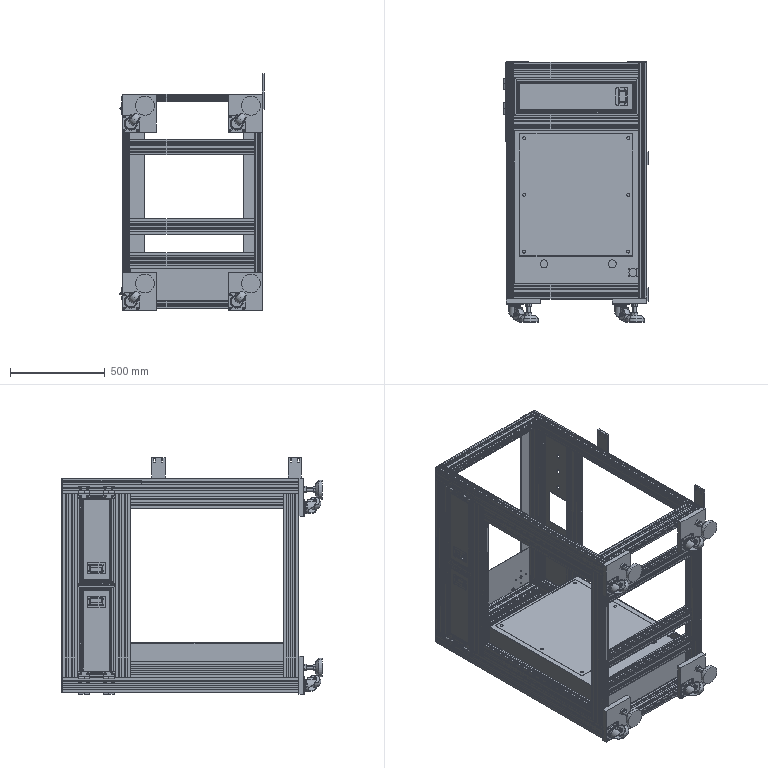Assembly | SolidWorks | mm | 62 component files | 97 solids | 3497 faces | box 762 x 1375 x 1252 mm | volume 33936133 mm3 | plane 2019 | cylinder 1170 | cone 148 | torus 128 | spline 24 | sphere 8 | commonest cylinder face diameters 8 x264 19 x216 6.8 x112 2 x60 10 x56 7 x56 5.5 x48 20 x32
Bill of materials:
10-15A | 1 |  | Long, narrow flat bar with small clipped corners and four through-holes arranged symmetrically along its length.
AluminumAlloyDoorAcrylicPlate(RearDoor) | 1 |  | Flat rectangular panel made of two stacked layers, with two hinge-like tabs along one short edge and a raised rounded-rectangle boss near the other end.
AluminumAlloyDoorAcrylicPlate(UpperSmallDoor) | 1 |  | Tall rectangular panel with hinge-like tabs at both short ends and two raised rounded-rectangle bosses near mid-height. It appears to be two panel sections stacked end to end.
EF4080-1080 | 1 |  | Straight extruded-style bar with a rectangular, multi-slot cross-section, shown standing vertically.
EF4080-500 | 4 |  | Long straight bar with the same kind of rectangular multi-slot cross-section, shown lying diagonally.
EF4080-550 | 2 |  | Long straight slotted bar whose cross-section looks the same as parts 3 and 4.
EF4080-920 | 5 |  | Straight slotted bar with a rectangular multi-cavity cross-section, shown standing vertically.
EF4080-940 | 8 |  | Long straight bar with a rectangular slotted cross-section, shown lying flat, with slots along the top face and the sides.
DistributionBox1 | 1 |  | Rectangular box-shaped body with plain faces. Holes are grouped near one edge of the top face, and there is one hole in a side face.
DistributionBoxDoor | 2 |  | Thin flat rectangular plate with no visible holes or features.
ElectricalControlPanel | 1 |  | Shallow square tray: a flat plate with a low upturned rim on all four edges and six small through-holes.
FrontSealingPlate | 1 |  | Long rectangular plate with short flanges bent along both long edges, forming a shallow channel.
TouchScreenPanel | 1 |  | Long, narrow rectangular flat plate. It has five small round through-holes on its centerline (three above and two below) and one rectangular through-cutout between the two groups.
CJH65bearing-322 | 4 |  | Solid cylinder whose length is roughly twice its diameter. Each end face shows a smaller concentric circular region, which suggests an edge chamfer/round, a shallow recess, or a boss.
CJH65body-322 | 4 |  | Compound fitting-like body. A cylindrical cup/socket with a large rounded closed end is joined at the side to an open, rectangular, channel-like clamp section. A bolt with hex head and nut is visible across the clamp section's slot.
CJH65swivel-322 | 4 |  | Square flat flange plate with rounded corners and four round through-holes, one near each corner. A central circular feature projects from one face, with tapered side walls and a flat top.
CJH65wheel-322 | 4 |  | Barrel-shaped body: a sphere-like or convex outer surface truncated by two parallel flat end faces, with a central cylindrical through-bore along the axis.
FBR20nut-322 | 4 |  | Hexagonal prism with a central round through-bore. The corners are chamfered on one end face, giving the curved chamfer arcs typical of a hex nut form.
pad1100-20-100pad1-322 | 4 |  | Disc-shaped base whose upper rim is conically tapered. On top sits a small hexagonal section, from which a long, slender cylindrical rod extends along the axis. The overall shape resembles a leveling foot.
WheelFixingPlate-322 | 4 |  | Thick, nearly square rectangular plate with five round through-holes: one larger hole near an upper corner region and four smaller holes in a rectangular/square pattern toward the opposite side.
30-42A | 1 |  | Very thin, large rectangular sheet with many round through-holes of several sizes. These include small holes near the edges and corners, two medium holes, and a cluster of one central hole surrounded by four tiny holes.
30-43A | 1 |  | Long, very thin rectangular strip with four small round through-holes, evenly spaced in a line near one long edge.
30-44A | 1 |  | Long, very thin rectangular strip with four small round through-holes, evenly spaced in a line near one long edge (the side opposite to the similar strip in the set).
30-71A | 2 |  | Thick rectangular plate. Two parallel elongated slots with rounded ends run lengthwise at one end, and four round through-holes form a two-by-two pattern at the other end.
Mates:
1. coincident | 30-01A-1/EF4080-920-4 face at (-423.23, 712.155, -40) dir (0, 1, 0) | 30-43A-1 face at (-447.43, 712.155, 40) dir (0, -1, 0)
2. coincident | 30-01A-1/EF4080-500-1 face at (-447.43, 712.155, 40) dir (0, 0, 1) | 30-43A-1 face at (-327.43, 712.155, 40) dir (0, 0, 1)
3. coincident | 30-01A-1/EF4080-500-1 face at (-447.43, 712.155, 40) dir (-1, 0, 0) | 30-43A-1 face at (-447.43, 712.155, 40) dir (-1, 0, 0)
4. coincident | 30-01A-1/EF4080-920-3 face at (276.77, 712.155, -40) dir (0, 1, 0) | 30-44A-1 face at (192.57, 712.155, 40) dir (0, -1, 0)
5. coincident | 30-01A-1/EF4080-500-2 face at (292.57, 712.155, -15.8) dir (1, 0, 0) | 30-44A-1 face at (292.57, 712.155, 40) dir (1, 0, 0)
6. coincident | 30-01A-1/EF4080-500-2 face at (276.77, 712.155, 40) dir (0, 0, 1) | 30-44A-1 face at (292.57, 712.155, 40) dir (0, 0, 1)
7. coincident | 30-01A-1/EF4080-940-6 face at (-407.43, 712.155, -1074.2) dir (0, 1, 0) | 30-42A-1 face at (-447.43, 712.155, -828) dir (0, -1, 0)
8. coincident | 30-01A-1/EF4080-500-4 face at (292.57, 712.155, -1090) dir (1, 0, 0) | 30-42A-1 face at (292.57, 714.155, -1090) dir (1, 0, 0)
9. coincident | 30-01A-1/EF4080-500-4 face at (276.77, 712.155, -1090) dir (0, 0, -1) | 30-42A-1 face at (-447.43, 714.155, -1090) dir (0, 0, -1)
10. coincident | 30-01A-1/EF4080-500-2 face at (292.57, 712.155, -15.8) dir (1, 0, 0) | 30-71A-1 face at (292.57, -480.845, -40) dir (-1, 0, 0)
11. coincident | 30-01A-1/EF4080-500-2 face at (276.77, 712.155, -40) dir (0, 0, -1) | 30-71A-1 face at (292.57, -480.845, -40) dir (0, 0, -1)
12. distance | 30-01A-1/EF4080-920-2 face at (276.77, -537.845, -40) dir (0, -1, 0) | 30-71A-1 face at (292.57, -550.845, 150) dir (0, -1, 0)
13. coincident | 30-01A-1/EF4080-500-1 face at (-447.43, 712.155, 15.8) dir (-1, 0, 0) | 10-15A-1 face at (-447.43, 712.155, 30) dir (1, 0, 0)
14. coincident | 30-01A-1/EF4080-940-7 face at (-407.43, 712.155, 40) dir (0, 1, 0) | 10-15A-1 face at (-449.43, 712.155, 30) dir (0, 1, 0)
15. distance | 30-01A-1/EF4080-500-1 face at (-447.43, 712.155, 40) dir (0, 0, 1) | 10-15A-1 face at (-449.43, 292.155, 10) dir (0, 0, -1)
16. coincident | EF4080-500-1 face at (-122.809, 641.189, -15.8) dir (1, 0, 0) | EF4080-940-1 face at (-122.809, -533.311, 20) dir (-1, 0, 0)
17. coincident | EF4080-500-1 face at (-138.609, 641.189, -40) dir (0, 0, -1) | EF4080-920-1 face at (-142.809, -604.311, -40) dir (0, 0, 1)
18. coincident | EF4080-500-1 face at (-122.809, 641.189, -40) dir (1, 0, 0) | EF4080-920-1 face at (-122.809, -553.011, -40) dir (1, 0, 0)
19. coincident | EF4080-500-1 face at (-142.809, -608.811, 35.5) dir (0, -1, 0) | EF4080-920-1 face at (-138.609, -608.811, -40) dir (0, -1, 0)
20. coincident | EF4080-500-1 face at (-138.609, 641.189, 40) dir (0, 0, 1) | EF4080-940-1 face at (-122.809, -553.011, 40) dir (0, 0, 1)
21. coincident | EF4080-500-1 face at (-142.809, -608.811, 35.5) dir (0, -1, 0) | EF4080-940-1 face at (-122.809, -608.811, 40) dir (0, -1, 0)
22. coincident | EF4080-500-3 face at (-122.809, 641.189, -1065.8) dir (1, 0, 0) | EF4080-940-5 face at (-122.809, -533.311, -1070) dir (-1, 0, 0)
23. coincident | EF4080-500-3 face at (-142.809, -608.811, -1014.5) dir (0, -1, 0) | EF4080-940-5 face at (-122.809, -608.811, -1050) dir (0, -1, 0)
24. coincident | EF4080-500-3 face at (-138.609, 641.189, -1090) dir (0, 0, -1) | EF4080-940-5 face at (-122.809, -584.611, -1090) dir (0, 0, -1)
25. coincident | EF4080-500-2 face at (561.391, 641.189, -40) dir (0, 0, -1) | EF4080-920-2 face at (557.191, -604.311, -40) dir (0, 0, 1)
26. coincident | EF4080-500-2 face at (577.191, 641.189, -40) dir (1, 0, 0) | EF4080-920-2 face at (577.191, -608.811, -40) dir (1, 0, 0)
27. coincident | EF4080-500-2 face at (557.191, -608.811, 35.5) dir (0, -1, 0) | EF4080-920-2 face at (561.391, -608.811, -40) dir (0, -1, 0)
28. coincident | EF4080-920-2 face at (537.191, -608.811, -40) dir (0, -1, 0) | Wheel-322-1/WheelFixingPlate-322-1 face at (577.191, -608.811, 40) dir (0, 1, 0)
29. coincident | EF4080-920-2 face at (577.191, -553.011, -40) dir (1, 0, 0) | Wheel-322-1/WheelFixingPlate-322-1 face at (577.191, -608.811, 40) dir (1, 0, 0)
30. coincident | EF4080-940-1 face at (-122.809, -553.011, 40) dir (0, 0, 1) | Wheel-322-1/WheelFixingPlate-322-1 face at (397.191, -608.811, 40) dir (0, 0, 1)
31. coincident | EF4080-920-2 face at (537.191, -584.611, -40) dir (-1, 0, 0) | EF4080-940-9 face at (537.191, -548.811, -273.5) dir (1, 0, 0)
32. coincident | EF4080-920-2 face at (537.191, -528.811, -40) dir (0, 1, 0) | EF4080-940-9 face at (-122.809, -528.811, -253.8) dir (0, 1, 0)
33. distance | EF4080-500-2 face at (537.191, 641.189, -40) dir (0, 0, -1) | EF4080-940-9 face at (-122.809, -528.811, -198) dir (0, 0, 1)
34. coincident | EF4080-500-2 face at (577.191, 641.189, -15.8) dir (1, 0, 0) | TouchScreenPanel-1 face at (577.191, 361.189, -40) dir (1, 0, 0)
35. coincident | EF4080-500-2 face at (561.391, 641.189, -40) dir (0, 0, -1) | TouchScreenPanel-1 face at (575.191, 361.189, -40) dir (0, 0, 1)
36. coincident | EF4080-920-3 face at (561.391, 561.189, -40) dir (0, -1, 0) | TouchScreenPanel-1 face at (575.191, 561.189, -40) dir (0, 1, 0)
37. coincident | EF4080-920-4 face at (-162.809, 561.189, -40) dir (-1, 0, 0) | AluminumAlloyDoorAcrylicPlate(UpperSmallDoor)-1 face at (-162.809, 531.189, -524) dir (-1, 0, 0)
38. coincident | EF4080-920-4 face at (-162.809, 561.189, -40) dir (0, -1, 0) | AluminumAlloyDoorAcrylicPlate(UpperSmallDoor)-1 face at (-162.809, 561.189, -524) dir (0, 1, 0)
39. coincident | EF4080-500-1 face at (-138.609, 641.189, -40) dir (0, 0, -1) | AluminumAlloyDoorAcrylicPlate(UpperSmallDoor)-1 face at (-154.059, 561.189, -40) dir (0, 0, 1)
40. coincident | EF4080-940-6 face at (-122.809, 561.189, -1090) dir (0, 0, -1) | AluminumAlloyDoorAcrylicPlate(RearDoor)-1 face at (537.191, 361.189, -1090) dir (0, 0, -1)
41. coincident | EF4080-940-10 face at (-122.809, -528.811, -673.8) dir (0, 1, 0) | FrontSealingPlate-1 face at (537.191, -528.811, -1050) dir (0, 1, 0)
42. coincident | EF4080-920-1 face at (-122.809, -553.011, -40) dir (1, 0, 0) | FrontSealingPlate-1 face at (-122.809, -530.811, -1050) dir (-1, 0, 0)
43. coincident | FrontSealingPlate-1 face at (537.191, -548.811, -878) dir (0, 0, 1) | EF4080-940-12 face at (-122.809, -553.011, -878) dir (0, 0, -1)
44. coincident | EF4080-500-3 face at (-162.809, 641.189, -1010) dir (0, 0, 1) | EF4080-550-1 face at (-162.809, 281.189, -1010) dir (0, 0, -1)
45. coincident | EF4080-500-1 face at (-138.609, 641.189, -40) dir (0, 0, -1) | EF4080-1080-1 face at (-142.809, 356.689, -40) dir (0, 0, 1)
46. coincident | EF4080-500-1 face at (-162.809, 641.189, 15.8) dir (-1, 0, 0) | EF4080-1080-1 face at (-162.809, 336.989, -1010) dir (-1, 0, 0)
47. coincident | EF4080-1080-1 face at (-162.809, 361.189, -1010) dir (0, 1, 0) | AluminumAlloyDoorAcrylicPlate(UpperSmallDoor)-1 face at (-161.559, 361.189, -524) dir (0, -1, 0)
48. coincident | EF4080-500-1 face at (-162.809, 641.189, -40) dir (0, 0, -1) | EF4080-550-2 face at (-162.809, 281.189, -40) dir (0, 0, 1)
49. coincident | EF4080-1080-1 face at (-162.809, 296.989, -1010) dir (-1, 0, 0) | EF4080-550-2 face at (-162.809, 281.189, -64.2) dir (-1, 0, 0)
50. coincident | EF4080-1080-1 face at (-138.609, 281.189, -1010) dir (0, -1, 0) | EF4080-550-2 face at (-142.809, 281.189, -44.5) dir (0, 1, 0)
51. coincident | EF4080-500-3 face at (-162.809, 641.189, -1034.2) dir (-1, 0, 0) | EF4080-550-1 face at (-162.809, 281.189, -954.2) dir (-1, 0, 0)
52. coincident | EF4080-920-1 face at (-162.809, -528.811, -40) dir (0, 1, 0) | EF4080-550-1 face at (-142.809, -528.811, -934.5) dir (0, -1, 0)
53. coincident | EF4080-940-12 face at (-122.809, -528.811, -853.8) dir (0, 1, 0) | ElectricalControlBox-1/DistributionBox1-1 face at (537.191, -528.811, -1090) dir (0, -1, 0)
54. coincident | EF4080-500-4 face at (537.191, 641.189, -1034.2) dir (-1, 0, 0) | ElectricalControlBox-1/DistributionBox1-1 face at (537.191, 281.189, -1090) dir (1, 0, 0)
55. coincident | EF4080-500-4 face at (537.191, 641.189, -1090) dir (0, 0, -1) | ElectricalControlBox-1/DistributionBoxDoor-1 face at (526.191, -517.811, -1090) dir (0, 0, -1)
56. coincident | EF4080-500-4 face at (537.191, 641.189, -1034.2) dir (-1, 0, 0) | AluminumAlloyDoorAcrylicPlate(RearDoor)-1 face at (537.191, 561.189, -1088.75) dir (1, 0, 0)
57. coincident | EF4080-940-6 face at (-122.809, 561.189, -1074.2) dir (0, -1, 0) | AluminumAlloyDoorAcrylicPlate(RearDoor)-1 face at (537.191, 561.189, -1090) dir (0, 1, 0)
58. coincident | DistributionBox1-1 face at (-445.975, -410.986, 260) dir (0, 0, 1) | DistributionBoxDoor-1 face at (-434.975, -399.986, 260) dir (0, 0, 1)
59. coincident | DistributionBox1-1 face at (-119.975, 388.014, 258) dir (0, -1, 0) | DistributionBoxDoor-1 face at (-434.975, 388.014, 260) dir (0, 1, 0)
60. coincident | DistributionBox1-1 face at (-434.975, 388.014, 250) dir (1, 0, 0) | DistributionBoxDoor-1 face at (-434.975, 388.014, 260) dir (-1, 0, 0)
61. coincident | DistributionBoxDoor-1 face at (-434.975, -399.986, 260) dir (0, 0, 1) | DistributionBoxDoor-2 face at (203.025, 388.014, 260) dir (0, 0, 1)
62. coincident | DistributionBox1-1 face at (-119.975, 388.014, 258) dir (0, -1, 0) | DistributionBoxDoor-2 face at (203.025, 388.014, 260) dir (0, 1, 0)
63. coincident | DistributionBox1-1 face at (203.025, -399.986, 250) dir (-1, 0, 0) | DistributionBoxDoor-2 face at (203.025, -399.986, 260) dir (1, 0, 0)
64. coincident | DistributionBox1-1 face at (-445.975, -410.986, 2) dir (0, 0, 1) | ElectricalControlPanel-1 face at (184.025, 384.014, 2) dir (0, 0, -1)
65. concentric | DistributionBox1-1 face at (-390.975, 359.014, 32) dir (0, 0, -1) r 4 | ElectricalControlPanel-1 face at (-390.975, 359.014, 12) dir (0, 0, 1) r 4.5
66. concentric | DistributionBox1-1 face at (159.025, 359.014, 32) dir (0, 0, -1) r 4 | ElectricalControlPanel-1 face at (159.025, 359.014, 12) dir (0, 0, 1) r 4.5
67. coincident | WheelFixingPlate-322-1 face at (-82.9, -50.745, -12.5) dir (0, 0, -1) | CJH65-322-1/CJH65swivel-322-1 face at (36.1, 48.255, -12.5) dir (0, 0, 1)
68. concentric | WheelFixingPlate-322-1 face at (107.1, 119.255, 12.5) dir (0, 0, 1) r 3.4 | CJH65-322-1/CJH65swivel-322-1 face at (107.1, 119.255, -15.7) dir (0, 0, 1) r 5.25
69. concentric | WheelFixingPlate-322-1 face at (107.1, 48.255, 12.5) dir (0, 0, 1) r 3.4 | CJH65-322-1/CJH65swivel-322-1 face at (107.1, 48.255, -15.7) dir (0, 0, 1) r 5.25
70. concentric | WheelFixingPlate-322-1 face at (-22.9, 9.255, 12.5) dir (0, 0, 1) r 10 | FBR100-20-322-1/pad1100-20-100pad1-322-1 face at (-22.9, 9.255, -110.5) dir (0, 0, 1) r 10
71. coincident | WheelFixingPlate-322-1 face at (-82.9, -50.745, -12.5) dir (0, 0, -1) | FBR100-20-322-1/FBR20nut-322-1 face at (-15.613, 25.713, -12.5) dir (0, 0, 1)
72. coincident | CJH65swivel-322-1 plane at (0, -9.6, 0) dir (0, 1, 0) | CJH65body-322-1 plane at (0, -9.6, 0) dir (0, 1, 0)
73. coincident | CJH65swivel-322-1 axis at (0, 50, 0) dir (0, -1, 0) | CJH65body-322-1 axis at (0, 50, 0) dir (0, -1, 0)
74. coincident | CJH65body-322-1 plane at (0, 0, 0) dir (0.641, 0, 0.7676) | CJH65bearing-322-1 plane at (-23.027, -59.5, 19.23) dir (-0.641, 0, -0.7676)
75. coincident | CJH65body-322-1 axis at (28.829, -59.5, 81.325) dir (-0.641, 0, -0.7676) | CJH65bearing-322-1 axis at (-74.882, -59.5, -42.866) dir (0.641, 0, 0.7676)
76. distance | CJH65bearing-322-1 plane at (-23.027, -59.5, 19.23) dir (-0.641, 0, -0.7676) | CJH65wheel-322-1 plane at (-23.027, -59.5, 19.23) dir (0.641, 0, 0.7676)
77. coincident | CJH65bearing-322-1 axis at (-74.882, -59.5, -42.866) dir (0.641, 0, 0.7676) | CJH65wheel-322-1 axis at (28.829, -59.5, 81.325) dir (-0.641, 0, -0.7676)
78. angle | CJH65bearing-322-1 plane at (-23.027, -59.5, 19.23) dir (0.006155, -1, -0.00514) | CJH65wheel-322-1 plane at (-23.027, -59.5, 19.23) dir (0.006155, -1, -0.00514)
79. coincident | pad1100-20-100pad1-322-1 axis at (0, 50, 0) dir (0, -1, 0) | FBR20nut-322-1 axis at (0, 48, 0) dir (0, 1, 0)
80. distance | FBR20nut-322-1 face at (17.674, 98, -3.408) dir (0, 1, 0) | pad1100-20-100pad1-322-1 face at (10, 48, 0) dir (0, 1, 0)